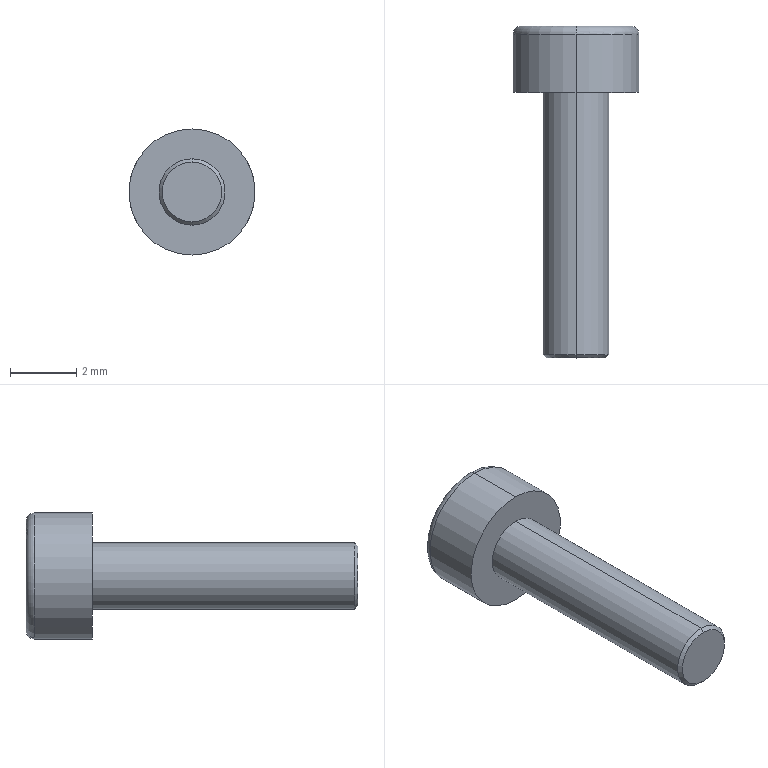Component | SolidWorks | hexagon socket head cap screws gb-4 | 1 solid | 25 faces | box 3.8 x 10 x 3.8 mm | volume 45 mm3 | plane 15 | cone 4 | cylinder 4 | torus 2 | commonest cylinder face diameters 2 x2 3.8 x2
STEP:
#1=COLOUR_RGB('',0.7922,0.8196,0.9333);
#2=FILL_AREA_STYLE_COLOUR('',#1);
#3=FILL_AREA_STYLE('',(#2));
#4=SURFACE_STYLE_FILL_AREA(#3);
#5=SURFACE_SIDE_STYLE('',(#4));
#6=SURFACE_STYLE_USAGE(.BOTH.,#5);
#7=PRESENTATION_STYLE_ASSIGNMENT((#6));
#8=CARTESIAN_POINT('',(1.349,0.4924,7.451));
#9=VERTEX_POINT('',#8);
#10=CARTESIAN_POINT('',(1.349,0.4924,7.522));
#11=VERTEX_POINT('',#10);
#12=CARTESIAN_POINT('',(1.349,0.4924,7.487));
#13=DIRECTION('',(0.,-1.,0.));
#14=DIRECTION('',(0.,0.,-1.));
#15=AXIS2_PLACEMENT_3D('',#12,#13,#14);
#16=CIRCLE('',#15,0.03543);
#17=EDGE_CURVE('',#9,#11,#16,.T.);
#18=ORIENTED_EDGE('',*,*,#17,.F.);
#19=CARTESIAN_POINT('',(1.349,0.4963,7.448));
#20=VERTEX_POINT('',#19);
#21=CARTESIAN_POINT('',(1.349,0.4924,7.451));
#22=DIRECTION('',(0.,0.7071,-0.7071));
#23=VECTOR('',#22,39.37);
#24=LINE('',#21,#23);
#25=EDGE_CURVE('',#9,#20,#24,.T.);
#26=ORIENTED_EDGE('',*,*,#25,.T.);
#27=CARTESIAN_POINT('',(1.349,0.4963,7.526));
#28=VERTEX_POINT('',#27);
#29=CARTESIAN_POINT('',(1.349,0.4963,7.487));
#30=DIRECTION('',(0.,1.,0.));
#31=DIRECTION('',(0.,0.,-1.));
#32=AXIS2_PLACEMENT_3D('',#29,#30,#31);
#33=CIRCLE('',#32,0.03937);
#34=EDGE_CURVE('',#28,#20,#33,.T.);
#35=ORIENTED_EDGE('',*,*,#34,.F.);
#36=CARTESIAN_POINT('',(1.349,0.4924,7.522));
#37=DIRECTION('',(0.,0.7071,0.7071));
#38=VECTOR('',#37,39.37);
#39=LINE('',#36,#38);
#40=EDGE_CURVE('',#11,#28,#39,.T.);
#41=ORIENTED_EDGE('',*,*,#40,.F.);
#42=EDGE_LOOP('',(#18,#26,#35,#41));
#43=FACE_OUTER_BOUND('',#42,.T.);
#44=CARTESIAN_POINT('',(1.349,0.4924,7.487));
#45=DIRECTION('',(0.,1.,0.));
#46=DIRECTION('',(0.,0.,1.));
#47=AXIS2_PLACEMENT_3D('',#44,#45,#46);
#48=CONICAL_SURFACE('',#47,0.03543,0.7854);
#49=ADVANCED_FACE('',(#43),#48,.T.);
#50=CARTESIAN_POINT('',(1.349,0.8861,7.552));
#51=VERTEX_POINT('',#50);
#52=CARTESIAN_POINT('',(1.349,0.8861,7.422));
#53=VERTEX_POINT('',#52);
#54=CARTESIAN_POINT('',(1.349,0.8861,7.487));
#55=DIRECTION('',(0.,1.,0.));
#56=DIRECTION('',(0.,0.,-1.));
#57=AXIS2_PLACEMENT_3D('',#54,#55,#56);
#58=CIRCLE('',#57,0.06496);
#59=EDGE_CURVE('',#51,#53,#58,.T.);
#60=ORIENTED_EDGE('',*,*,#59,.F.);
#61=CARTESIAN_POINT('',(1.349,0.8762,7.562));
#62=VERTEX_POINT('',#61);
#63=CARTESIAN_POINT('',(1.349,0.8762,7.552));
#64=DIRECTION('',(1.,0.,-0.));
#65=DIRECTION('',(0.,0.,-1.));
#66=AXIS2_PLACEMENT_3D('',#63,#64,#65);
#67=CIRCLE('',#66,0.009843);
#68=EDGE_CURVE('',#51,#62,#67,.T.);
#69=ORIENTED_EDGE('',*,*,#68,.T.);
#70=CARTESIAN_POINT('',(1.349,0.8762,7.412));
#71=VERTEX_POINT('',#70);
#72=CARTESIAN_POINT('',(1.349,0.8762,7.487));
#73=DIRECTION('',(0.,-1.,0.));
#74=DIRECTION('',(0.,0.,-1.));
#75=AXIS2_PLACEMENT_3D('',#72,#73,#74);
#76=CIRCLE('',#75,0.0748);
#77=EDGE_CURVE('',#71,#62,#76,.T.);
#78=ORIENTED_EDGE('',*,*,#77,.F.);
#79=CARTESIAN_POINT('',(1.349,0.8762,7.422));
#80=DIRECTION('',(-1.,0.,0.));
#81=DIRECTION('',(0.,0.,1.));
#82=AXIS2_PLACEMENT_3D('',#79,#80,#81);
#83=CIRCLE('',#82,0.009843);
#84=EDGE_CURVE('',#53,#71,#83,.T.);
#85=ORIENTED_EDGE('',*,*,#84,.F.);
#86=EDGE_LOOP('',(#60,#69,#78,#85));
#87=FACE_OUTER_BOUND('',#86,.T.);
#88=CARTESIAN_POINT('',(1.349,0.8762,7.487));
#89=DIRECTION('',(0.,-1.,0.));
#90=DIRECTION('',(0.,0.,-1.));
#91=AXIS2_PLACEMENT_3D('',#88,#89,#90);
#92=TOROIDAL_SURFACE('',#91,0.06496,0.009843);
#93=ADVANCED_FACE('',(#87),#92,.T.);
#94=CARTESIAN_POINT('',(1.349,0.8297,7.487));
#95=VERTEX_POINT('',#94);
#96=CARTESIAN_POINT('',(1.349,0.8467,7.516));
#97=VERTEX_POINT('',#96);
#98=CARTESIAN_POINT('',(1.349,0.8467,7.516));
#99=DIRECTION('',(0.,0.5,0.866));
#100=VECTOR('',#99,39.37);
#101=LINE('',#98,#100);
#102=EDGE_CURVE('',#95,#97,#101,.T.);
#103=ORIENTED_EDGE('',*,*,#102,.F.);
#104=CARTESIAN_POINT('',(1.349,0.8467,7.457));
#105=VERTEX_POINT('',#104);
#106=CARTESIAN_POINT('',(1.349,0.8467,7.457));
#107=DIRECTION('',(0.,0.5,-0.866));
#108=VECTOR('',#107,39.37);
#109=LINE('',#106,#108);
#110=EDGE_CURVE('',#95,#105,#109,.T.);
#111=ORIENTED_EDGE('',*,*,#110,.T.);
#112=CARTESIAN_POINT('',(1.334,0.8467,7.461));
#113=VERTEX_POINT('',#112);
#114=CARTESIAN_POINT('',(1.349,0.8467,7.487));
#115=DIRECTION('',(0.,1.,0.));
#116=DIRECTION('',(0.,0.,-1.));
#117=AXIS2_PLACEMENT_3D('',#114,#115,#116);
#118=CIRCLE('',#117,0.02953);
#119=EDGE_CURVE('',#105,#113,#118,.T.);
#120=ORIENTED_EDGE('',*,*,#119,.T.);
#121=CARTESIAN_POINT('',(1.32,0.8467,7.487));
#122=VERTEX_POINT('',#121);
#123=CARTESIAN_POINT('',(1.349,0.8467,7.487));
#124=DIRECTION('',(0.,1.,0.));
#125=DIRECTION('',(0.,0.,-1.));
#126=AXIS2_PLACEMENT_3D('',#123,#124,#125);
#127=CIRCLE('',#126,0.02953);
#128=EDGE_CURVE('',#113,#122,#127,.T.);
#129=ORIENTED_EDGE('',*,*,#128,.T.);
#130=CARTESIAN_POINT('',(1.334,0.8467,7.512));
#131=VERTEX_POINT('',#130);
#132=CARTESIAN_POINT('',(1.349,0.8467,7.487));
#133=DIRECTION('',(0.,1.,0.));
#134=DIRECTION('',(0.,0.,-1.));
#135=AXIS2_PLACEMENT_3D('',#132,#133,#134);
#136=CIRCLE('',#135,0.02953);
#137=EDGE_CURVE('',#122,#131,#136,.T.);
#138=ORIENTED_EDGE('',*,*,#137,.T.);
#139=CARTESIAN_POINT('',(1.349,0.8467,7.487));
#140=DIRECTION('',(0.,1.,0.));
#141=DIRECTION('',(0.,0.,-1.));
#142=AXIS2_PLACEMENT_3D('',#139,#140,#141);
#143=CIRCLE('',#142,0.02953);
#144=EDGE_CURVE('',#131,#97,#143,.T.);
#145=ORIENTED_EDGE('',*,*,#144,.T.);
#146=EDGE_LOOP('',(#103,#111,#120,#129,#138,#145));
#147=FACE_OUTER_BOUND('',#146,.T.);
#148=CARTESIAN_POINT('',(1.349,0.8467,7.487));
#149=DIRECTION('',(0.,1.,0.));
#150=DIRECTION('',(0.,0.,1.));
#151=AXIS2_PLACEMENT_3D('',#148,#149,#150);
#152=CONICAL_SURFACE('',#151,0.02953,1.047);
#153=ADVANCED_FACE('',(#147),#152,.F.);
#154=ORIENTED_EDGE('',*,*,#34,.T.);
#155=CARTESIAN_POINT('',(1.349,0.8073,7.448));
#156=VERTEX_POINT('',#155);
#157=CARTESIAN_POINT('',(1.349,0.4924,7.448));
#158=DIRECTION('',(0.,1.,0.));
#159=VECTOR('',#158,39.37);
#160=LINE('',#157,#159);
#161=EDGE_CURVE('',#20,#156,#160,.T.);
#162=ORIENTED_EDGE('',*,*,#161,.T.);
#163=CARTESIAN_POINT('',(1.349,0.8073,7.526));
#164=VERTEX_POINT('',#163);
#165=CARTESIAN_POINT('',(1.349,0.8073,7.487));
#166=DIRECTION('',(0.,-1.,0.));
#167=DIRECTION('',(0.,0.,-1.));
#168=AXIS2_PLACEMENT_3D('',#165,#166,#167);
#169=CIRCLE('',#168,0.03937);
#170=EDGE_CURVE('',#156,#164,#169,.T.);
#171=ORIENTED_EDGE('',*,*,#170,.T.);
#172=CARTESIAN_POINT('',(1.349,0.4924,7.526));
#173=DIRECTION('',(0.,1.,0.));
#174=VECTOR('',#173,39.37);
#175=LINE('',#172,#174);
#176=EDGE_CURVE('',#28,#164,#175,.T.);
#177=ORIENTED_EDGE('',*,*,#176,.F.);
#178=EDGE_LOOP('',(#154,#162,#171,#177));
#179=FACE_OUTER_BOUND('',#178,.T.);
#180=CARTESIAN_POINT('',(1.349,0.4924,7.487));
#181=DIRECTION('',(0.,1.,0.));
#182=DIRECTION('',(0.,0.,1.));
#183=AXIS2_PLACEMENT_3D('',#180,#181,#182);
#184=CYLINDRICAL_SURFACE('',#183,0.03937);
#185=ADVANCED_FACE('',(#179),#184,.T.);
#186=CARTESIAN_POINT('',(1.349,0.8073,7.412));
#187=VERTEX_POINT('',#186);
#188=CARTESIAN_POINT('',(1.349,0.8073,7.562));
#189=VERTEX_POINT('',#188);
#190=CARTESIAN_POINT('',(1.349,0.8073,7.487));
#191=DIRECTION('',(0.,-1.,0.));
#192=DIRECTION('',(0.,0.,-1.));
#193=AXIS2_PLACEMENT_3D('',#190,#191,#192);
#194=CIRCLE('',#193,0.0748);
#195=EDGE_CURVE('',#187,#189,#194,.T.);
#196=ORIENTED_EDGE('',*,*,#195,.F.);
#197=CARTESIAN_POINT('',(1.349,0.8073,7.412));
#198=DIRECTION('',(0.,1.,0.));
#199=VECTOR('',#198,39.37);
#200=LINE('',#197,#199);
#201=EDGE_CURVE('',#187,#71,#200,.T.);
#202=ORIENTED_EDGE('',*,*,#201,.T.);
#203=ORIENTED_EDGE('',*,*,#77,.T.);
#204=CARTESIAN_POINT('',(1.349,0.8073,7.562));
#205=DIRECTION('',(0.,1.,0.));
#206=VECTOR('',#205,39.37);
#207=LINE('',#204,#206);
#208=EDGE_CURVE('',#189,#62,#207,.T.);
#209=ORIENTED_EDGE('',*,*,#208,.F.);
#210=EDGE_LOOP('',(#196,#202,#203,#209));
#211=FACE_OUTER_BOUND('',#210,.T.);
#212=CARTESIAN_POINT('',(1.349,0.8073,7.487));
#213=DIRECTION('',(0.,1.,0.));
#214=DIRECTION('',(0.,0.,1.));
#215=AXIS2_PLACEMENT_3D('',#212,#213,#214);
#216=CYLINDRICAL_SURFACE('',#215,0.0748);
#217=ADVANCED_FACE('',(#211),#216,.T.);
#218=ORIENTED_EDGE('',*,*,#128,.F.);
#219=CARTESIAN_POINT('',(1.32,0.8467,7.47));
#220=VERTEX_POINT('',#219);
#221=CARTESIAN_POINT('',(1.32,0.8467,7.47));
#222=DIRECTION('',(0.866,0.,-0.5));
#223=VECTOR('',#222,39.37);
#224=LINE('',#221,#223);
#225=EDGE_CURVE('',#220,#113,#224,.T.);
#226=ORIENTED_EDGE('',*,*,#225,.F.);
#227=CARTESIAN_POINT('',(1.32,0.8467,7.504));
#228=DIRECTION('',(-0.,0.,-1.));
#229=VECTOR('',#228,39.37);
#230=LINE('',#227,#229);
#231=EDGE_CURVE('',#122,#220,#230,.T.);
#232=ORIENTED_EDGE('',*,*,#231,.F.);
#233=EDGE_LOOP('',(#218,#226,#232));
#234=FACE_OUTER_BOUND('',#233,.T.);
#235=CARTESIAN_POINT('',(1.349,0.8467,7.453));
#236=DIRECTION('',(0.,-1.,0.));
#237=DIRECTION('',(0.,0.,-1.));
#238=AXIS2_PLACEMENT_3D('',#235,#236,#237);
#239=PLANE('',#238);
#240=ADVANCED_FACE('',(#234),#239,.F.);
#241=ORIENTED_EDGE('',*,*,#137,.F.);
#242=CARTESIAN_POINT('',(1.32,0.8467,7.504));
#243=VERTEX_POINT('',#242);
#244=CARTESIAN_POINT('',(1.32,0.8467,7.504));
#245=DIRECTION('',(-0.,0.,-1.));
#246=VECTOR('',#245,39.37);
#247=LINE('',#244,#246);
#248=EDGE_CURVE('',#243,#122,#247,.T.);
#249=ORIENTED_EDGE('',*,*,#248,.F.);
#250=CARTESIAN_POINT('',(1.349,0.8467,7.521));
#251=DIRECTION('',(-0.866,0.,-0.5));
#252=VECTOR('',#251,39.37);
#253=LINE('',#250,#252);
#254=EDGE_CURVE('',#131,#243,#253,.T.);
#255=ORIENTED_EDGE('',*,*,#254,.F.);
#256=EDGE_LOOP('',(#241,#249,#255));
#257=FACE_OUTER_BOUND('',#256,.T.);
#258=CARTESIAN_POINT('',(1.349,0.8467,7.453));
#259=DIRECTION('',(0.,-1.,0.));
#260=DIRECTION('',(0.,0.,-1.));
#261=AXIS2_PLACEMENT_3D('',#258,#259,#260);
#262=PLANE('',#261);
#263=ADVANCED_FACE('',(#257),#262,.F.);
#264=ORIENTED_EDGE('',*,*,#144,.F.);
#265=CARTESIAN_POINT('',(1.349,0.8467,7.521));
#266=VERTEX_POINT('',#265);
#267=CARTESIAN_POINT('',(1.349,0.8467,7.521));
#268=DIRECTION('',(-0.866,0.,-0.5));
#269=VECTOR('',#268,39.37);
#270=LINE('',#267,#269);
#271=EDGE_CURVE('',#266,#131,#270,.T.);
#272=ORIENTED_EDGE('',*,*,#271,.F.);
#273=CARTESIAN_POINT('',(1.364,0.8467,7.512));
#274=VERTEX_POINT('',#273);
#275=CARTESIAN_POINT('',(1.379,0.8467,7.504));
#276=DIRECTION('',(-0.866,0.,0.5));
#277=VECTOR('',#276,39.37);
#278=LINE('',#275,#277);
#279=EDGE_CURVE('',#274,#266,#278,.T.);
#280=ORIENTED_EDGE('',*,*,#279,.F.);
#281=CARTESIAN_POINT('',(1.349,0.8467,7.487));
#282=DIRECTION('',(0.,1.,0.));
#283=DIRECTION('',(0.,0.,-1.));
#284=AXIS2_PLACEMENT_3D('',#281,#282,#283);
#285=CIRCLE('',#284,0.02953);
#286=EDGE_CURVE('',#97,#274,#285,.T.);
#287=ORIENTED_EDGE('',*,*,#286,.F.);
#288=EDGE_LOOP('',(#264,#272,#280,#287));
#289=FACE_OUTER_BOUND('',#288,.T.);
#290=CARTESIAN_POINT('',(1.349,0.8467,7.453));
#291=DIRECTION('',(0.,-1.,0.));
#292=DIRECTION('',(0.,0.,-1.));
#293=AXIS2_PLACEMENT_3D('',#290,#291,#292);
#294=PLANE('',#293);
#295=ADVANCED_FACE('',(#289),#294,.F.);
#296=CARTESIAN_POINT('',(1.379,0.8467,7.487));
#297=VERTEX_POINT('',#296);
#298=CARTESIAN_POINT('',(1.349,0.8467,7.487));
#299=DIRECTION('',(0.,1.,0.));
#300=DIRECTION('',(0.,0.,-1.));
#301=AXIS2_PLACEMENT_3D('',#298,#299,#300);
#302=CIRCLE('',#301,0.02953);
#303=EDGE_CURVE('',#274,#297,#302,.T.);
#304=ORIENTED_EDGE('',*,*,#303,.F.);
#305=CARTESIAN_POINT('',(1.379,0.8467,7.504));
#306=VERTEX_POINT('',#305);
#307=CARTESIAN_POINT('',(1.379,0.8467,7.504));
#308=DIRECTION('',(-0.866,0.,0.5));
#309=VECTOR('',#308,39.37);
#310=LINE('',#307,#309);
#311=EDGE_CURVE('',#306,#274,#310,.T.);
#312=ORIENTED_EDGE('',*,*,#311,.F.);
#313=CARTESIAN_POINT('',(1.379,0.8467,7.47));
#314=DIRECTION('',(0.,0.,1.));
#315=VECTOR('',#314,39.37);
#316=LINE('',#313,#315);
#317=EDGE_CURVE('',#297,#306,#316,.T.);
#318=ORIENTED_EDGE('',*,*,#317,.F.);
#319=EDGE_LOOP('',(#304,#312,#318));
#320=FACE_OUTER_BOUND('',#319,.T.);
#321=CARTESIAN_POINT('',(1.349,0.8467,7.453));
#322=DIRECTION('',(0.,-1.,0.));
#323=DIRECTION('',(0.,0.,-1.));
#324=AXIS2_PLACEMENT_3D('',#321,#322,#323);
#325=PLANE('',#324);
#326=ADVANCED_FACE('',(#320),#325,.F.);
#327=CARTESIAN_POINT('',(1.364,0.8467,7.461));
#328=VERTEX_POINT('',#327);
#329=CARTESIAN_POINT('',(1.349,0.8467,7.487));
#330=DIRECTION('',(0.,-1.,0.));
#331=DIRECTION('',(0.,0.,-1.));
#332=AXIS2_PLACEMENT_3D('',#329,#330,#331);
#333=CIRCLE('',#332,0.02953);
#334=EDGE_CURVE('',#328,#297,#333,.T.);
#335=ORIENTED_EDGE('',*,*,#334,.T.);
#336=CARTESIAN_POINT('',(1.379,0.8467,7.47));
#337=VERTEX_POINT('',#336);
#338=CARTESIAN_POINT('',(1.379,0.8467,7.47));
#339=DIRECTION('',(0.,0.,1.));
#340=VECTOR('',#339,39.37);
#341=LINE('',#338,#340);
#342=EDGE_CURVE('',#337,#297,#341,.T.);
#343=ORIENTED_EDGE('',*,*,#342,.F.);
#344=CARTESIAN_POINT('',(1.349,0.8467,7.453));
#345=DIRECTION('',(0.866,0.,0.5));
#346=VECTOR('',#345,39.37);
#347=LINE('',#344,#346);
#348=EDGE_CURVE('',#328,#337,#347,.T.);
#349=ORIENTED_EDGE('',*,*,#348,.F.);
#350=EDGE_LOOP('',(#335,#343,#349));
#351=FACE_OUTER_BOUND('',#350,.T.);
#352=CARTESIAN_POINT('',(1.349,0.8467,7.453));
#353=DIRECTION('',(0.,-1.,0.));
#354=DIRECTION('',(0.,0.,-1.));
#355=AXIS2_PLACEMENT_3D('',#352,#353,#354);
#356=PLANE('',#355);
#357=ADVANCED_FACE('',(#351),#356,.F.);
#358=CARTESIAN_POINT('',(1.349,0.8467,7.487));
#359=DIRECTION('',(0.,1.,0.));
#360=DIRECTION('',(0.,0.,-1.));
#361=AXIS2_PLACEMENT_3D('',#358,#359,#360);
#362=CIRCLE('',#361,0.02953);
#363=EDGE_CURVE('',#328,#105,#362,.T.);
#364=ORIENTED_EDGE('',*,*,#363,.F.);
#365=CARTESIAN_POINT('',(1.349,0.8467,7.453));
#366=VERTEX_POINT('',#365);
#367=CARTESIAN_POINT('',(1.349,0.8467,7.453));
#368=DIRECTION('',(0.866,0.,0.5));
#369=VECTOR('',#368,39.37);
#370=LINE('',#367,#369);
#371=EDGE_CURVE('',#366,#328,#370,.T.);
#372=ORIENTED_EDGE('',*,*,#371,.F.);
#373=CARTESIAN_POINT('',(1.32,0.8467,7.47));
#374=DIRECTION('',(0.866,0.,-0.5));
#375=VECTOR('',#374,39.37);
#376=LINE('',#373,#375);
#377=EDGE_CURVE('',#113,#366,#376,.T.);
#378=ORIENTED_EDGE('',*,*,#377,.F.);
#379=ORIENTED_EDGE('',*,*,#119,.F.);
#380=EDGE_LOOP('',(#364,#372,#378,#379));
#381=FACE_OUTER_BOUND('',#380,.T.);
#382=CARTESIAN_POINT('',(1.349,0.8467,7.453));
#383=DIRECTION('',(0.,-1.,0.));
#384=DIRECTION('',(0.,0.,-1.));
#385=AXIS2_PLACEMENT_3D('',#382,#383,#384);
#386=PLANE('',#385);
#387=ADVANCED_FACE('',(#381),#386,.F.);
#388=CARTESIAN_POINT('',(1.349,0.8861,7.487));
#389=DIRECTION('',(0.,1.,0.));
#390=DIRECTION('',(0.,0.,-1.));
#391=AXIS2_PLACEMENT_3D('',#388,#389,#390);
#392=CIRCLE('',#391,0.06496);
#393=EDGE_CURVE('',#53,#51,#392,.T.);
#394=ORIENTED_EDGE('',*,*,#393,.T.);
#395=ORIENTED_EDGE('',*,*,#59,.T.);
#396=EDGE_LOOP('',(#394,#395));
#397=FACE_OUTER_BOUND('',#396,.T.);
#398=CARTESIAN_POINT('',(1.32,0.8861,7.47));
#399=VERTEX_POINT('',#398);
#400=CARTESIAN_POINT('',(1.349,0.8861,7.453));
#401=VERTEX_POINT('',#400);
#402=CARTESIAN_POINT('',(1.32,0.8861,7.47));
#403=DIRECTION('',(0.866,0.,-0.5));
#404=VECTOR('',#403,39.37);
#405=LINE('',#402,#404);
#406=EDGE_CURVE('',#399,#401,#405,.T.);
#407=ORIENTED_EDGE('',*,*,#406,.T.);
#408=CARTESIAN_POINT('',(1.379,0.8861,7.47));
#409=VERTEX_POINT('',#408);
#410=CARTESIAN_POINT('',(1.349,0.8861,7.453));
#411=DIRECTION('',(0.866,0.,0.5));
#412=VECTOR('',#411,39.37);
#413=LINE('',#410,#412);
#414=EDGE_CURVE('',#401,#409,#413,.T.);
#415=ORIENTED_EDGE('',*,*,#414,.T.);
#416=CARTESIAN_POINT('',(1.379,0.8861,7.504));
#417=VERTEX_POINT('',#416);
#418=CARTESIAN_POINT('',(1.379,0.8861,7.47));
#419=DIRECTION('',(0.,0.,1.));
#420=VECTOR('',#419,39.37);
#421=LINE('',#418,#420);
#422=EDGE_CURVE('',#409,#417,#421,.T.);
#423=ORIENTED_EDGE('',*,*,#422,.T.);
#424=CARTESIAN_POINT('',(1.349,0.8861,7.521));
#425=VERTEX_POINT('',#424);
#426=CARTESIAN_POINT('',(1.379,0.8861,7.504));
#427=DIRECTION('',(-0.866,0.,0.5));
#428=VECTOR('',#427,39.37);
#429=LINE('',#426,#428);
#430=EDGE_CURVE('',#417,#425,#429,.T.);
#431=ORIENTED_EDGE('',*,*,#430,.T.);
#432=CARTESIAN_POINT('',(1.32,0.8861,7.504));
#433=VERTEX_POINT('',#432);
#434=CARTESIAN_POINT('',(1.349,0.8861,7.521));
#435=DIRECTION('',(-0.866,0.,-0.5));
#436=VECTOR('',#435,39.37);
#437=LINE('',#434,#436);
#438=EDGE_CURVE('',#425,#433,#437,.T.);
#439=ORIENTED_EDGE('',*,*,#438,.T.);
#440=CARTESIAN_POINT('',(1.32,0.8861,7.504));
#441=DIRECTION('',(-0.,0.,-1.));
#442=VECTOR('',#441,39.37);
#443=LINE('',#440,#442);
#444=EDGE_CURVE('',#433,#399,#443,.T.);
#445=ORIENTED_EDGE('',*,*,#444,.T.);
#446=EDGE_LOOP('',(#407,#415,#423,#431,#439,#445));
#447=FACE_BOUND('',#446,.T.);
#448=CARTESIAN_POINT('',(1.349,0.8861,7.487));
#449=DIRECTION('',(0.,-1.,0.));
#450=DIRECTION('',(0.,0.,-1.));
#451=AXIS2_PLACEMENT_3D('',#448,#449,#450);
#452=PLANE('',#451);
#453=ADVANCED_FACE('',(#397,#447),#452,.F.);
#454=CARTESIAN_POINT('',(1.349,0.8073,7.487));
#455=DIRECTION('',(0.,-1.,0.));
#456=DIRECTION('',(0.,0.,-1.));
#457=AXIS2_PLACEMENT_3D('',#454,#455,#456);
#458=CIRCLE('',#457,0.0748);
#459=EDGE_CURVE('',#189,#187,#458,.T.);
#460=ORIENTED_EDGE('',*,*,#459,.T.);
#461=ORIENTED_EDGE('',*,*,#195,.T.);
#462=EDGE_LOOP('',(#460,#461));
#463=FACE_OUTER_BOUND('',#462,.T.);
#464=CARTESIAN_POINT('',(1.349,0.8073,7.487));
#465=DIRECTION('',(0.,-1.,0.));
#466=DIRECTION('',(0.,0.,-1.));
#467=AXIS2_PLACEMENT_3D('',#464,#465,#466);
#468=CIRCLE('',#467,0.03937);
#469=EDGE_CURVE('',#164,#156,#468,.T.);
#470=ORIENTED_EDGE('',*,*,#469,.F.);
#471=ORIENTED_EDGE('',*,*,#170,.F.);
#472=EDGE_LOOP('',(#470,#471));
#473=FACE_BOUND('',#472,.T.);
#474=CARTESIAN_POINT('',(1.349,0.8073,7.487));
#475=DIRECTION('',(0.,-1.,0.));
#476=DIRECTION('',(0.,0.,-1.));
#477=AXIS2_PLACEMENT_3D('',#474,#475,#476);
#478=PLANE('',#477);
#479=ADVANCED_FACE('',(#463,#473),#478,.T.);
#480=ORIENTED_EDGE('',*,*,#201,.F.);
#481=ORIENTED_EDGE('',*,*,#459,.F.);
#482=ORIENTED_EDGE('',*,*,#208,.T.);
#483=CARTESIAN_POINT('',(1.349,0.8762,7.487));
#484=DIRECTION('',(0.,-1.,0.));
#485=DIRECTION('',(0.,0.,-1.));
#486=AXIS2_PLACEMENT_3D('',#483,#484,#485);
#487=CIRCLE('',#486,0.0748);
#488=EDGE_CURVE('',#62,#71,#487,.T.);
#489=ORIENTED_EDGE('',*,*,#488,.T.);
#490=EDGE_LOOP('',(#480,#481,#482,#489));
#491=FACE_OUTER_BOUND('',#490,.T.);
#492=CARTESIAN_POINT('',(1.349,0.8073,7.487));
#493=DIRECTION('',(0.,1.,0.));
#494=DIRECTION('',(0.,0.,1.));
#495=AXIS2_PLACEMENT_3D('',#492,#493,#494);
#496=CYLINDRICAL_SURFACE('',#495,0.0748);
#497=ADVANCED_FACE('',(#491),#496,.T.);
#498=ORIENTED_EDGE('',*,*,#161,.F.);
#499=CARTESIAN_POINT('',(1.349,0.4963,7.487));
#500=DIRECTION('',(0.,1.,0.));
#501=DIRECTION('',(0.,0.,-1.));
#502=AXIS2_PLACEMENT_3D('',#499,#500,#501);
#503=CIRCLE('',#502,0.03937);
#504=EDGE_CURVE('',#20,#28,#503,.T.);
#505=ORIENTED_EDGE('',*,*,#504,.T.);
#506=ORIENTED_EDGE('',*,*,#176,.T.);
#507=ORIENTED_EDGE('',*,*,#469,.T.);
#508=EDGE_LOOP('',(#498,#505,#506,#507));
#509=FACE_OUTER_BOUND('',#508,.T.);
#510=CARTESIAN_POINT('',(1.349,0.4924,7.487));
#511=DIRECTION('',(0.,1.,0.));
#512=DIRECTION('',(0.,0.,1.));
#513=AXIS2_PLACEMENT_3D('',#510,#511,#512);
#514=CYLINDRICAL_SURFACE('',#513,0.03937);
#515=ADVANCED_FACE('',(#509),#514,.T.);
#516=CARTESIAN_POINT('',(1.349,0.4924,7.487));
#517=DIRECTION('',(0.,-1.,0.));
#518=DIRECTION('',(0.,0.,-1.));
#519=AXIS2_PLACEMENT_3D('',#516,#517,#518);
#520=CIRCLE('',#519,0.03543);
#521=EDGE_CURVE('',#11,#9,#520,.T.);
#522=ORIENTED_EDGE('',*,*,#521,.T.);
#523=ORIENTED_EDGE('',*,*,#17,.T.);
#524=EDGE_LOOP('',(#522,#523));
#525=FACE_OUTER_BOUND('',#524,.T.);
#526=CARTESIAN_POINT('',(1.349,0.4924,7.487));
#527=DIRECTION('',(0.,-1.,0.));
#528=DIRECTION('',(0.,0.,-1.));
#529=AXIS2_PLACEMENT_3D('',#526,#527,#528);
#530=PLANE('',#529);
#531=ADVANCED_FACE('',(#525),#530,.T.);
#532=ORIENTED_EDGE('',*,*,#406,.F.);
#533=CARTESIAN_POINT('',(1.32,0.8467,7.47));
#534=DIRECTION('',(0.,1.,0.));
#535=VECTOR('',#534,39.37);
#536=LINE('',#533,#535);
#537=EDGE_CURVE('',#220,#399,#536,.T.);
#538=ORIENTED_EDGE('',*,*,#537,.F.);
#539=ORIENTED_EDGE('',*,*,#225,.T.);
#540=ORIENTED_EDGE('',*,*,#377,.T.);
#541=CARTESIAN_POINT('',(1.349,0.8467,7.453));
#542=DIRECTION('',(0.,1.,0.));
#543=VECTOR('',#542,39.37);
#544=LINE('',#541,#543);
#545=EDGE_CURVE('',#366,#401,#544,.T.);
#546=ORIENTED_EDGE('',*,*,#545,.T.);
#547=EDGE_LOOP('',(#532,#538,#539,#540,#546));
#548=FACE_OUTER_BOUND('',#547,.T.);
#549=CARTESIAN_POINT('',(1.32,0.8467,7.47));
#550=DIRECTION('',(0.5,0.,0.866));
#551=DIRECTION('',(-0.866,0.,0.5));
#552=AXIS2_PLACEMENT_3D('',#549,#550,#551);
#553=PLANE('',#552);
#554=ADVANCED_FACE('',(#548),#553,.T.);
#555=ORIENTED_EDGE('',*,*,#414,.F.);
#556=ORIENTED_EDGE('',*,*,#545,.F.);
#557=ORIENTED_EDGE('',*,*,#371,.T.);
#558=ORIENTED_EDGE('',*,*,#348,.T.);
#559=CARTESIAN_POINT('',(1.379,0.8467,7.47));
#560=DIRECTION('',(0.,1.,0.));
#561=VECTOR('',#560,39.37);
#562=LINE('',#559,#561);
#563=EDGE_CURVE('',#337,#409,#562,.T.);
#564=ORIENTED_EDGE('',*,*,#563,.T.);
#565=EDGE_LOOP('',(#555,#556,#557,#558,#564));
#566=FACE_OUTER_BOUND('',#565,.T.);
#567=CARTESIAN_POINT('',(1.349,0.8467,7.453));
#568=DIRECTION('',(-0.5,0.,0.866));
#569=DIRECTION('',(-0.866,0.,-0.5));
#570=AXIS2_PLACEMENT_3D('',#567,#568,#569);
#571=PLANE('',#570);
#572=ADVANCED_FACE('',(#566),#571,.T.);
#573=ORIENTED_EDGE('',*,*,#422,.F.);
#574=ORIENTED_EDGE('',*,*,#563,.F.);
#575=ORIENTED_EDGE('',*,*,#342,.T.);
#576=ORIENTED_EDGE('',*,*,#317,.T.);
#577=CARTESIAN_POINT('',(1.379,0.8467,7.504));
#578=DIRECTION('',(0.,1.,0.));
#579=VECTOR('',#578,39.37);
#580=LINE('',#577,#579);
#581=EDGE_CURVE('',#306,#417,#580,.T.);
#582=ORIENTED_EDGE('',*,*,#581,.T.);
#583=EDGE_LOOP('',(#573,#574,#575,#576,#582));
#584=FACE_OUTER_BOUND('',#583,.T.);
#585=CARTESIAN_POINT('',(1.379,0.8467,7.47));
#586=DIRECTION('',(-1.,0.,0.));
#587=DIRECTION('',(0.,0.,-1.));
#588=AXIS2_PLACEMENT_3D('',#585,#586,#587);
#589=PLANE('',#588);
#590=ADVANCED_FACE('',(#584),#589,.T.);
#591=ORIENTED_EDGE('',*,*,#430,.F.);
#592=ORIENTED_EDGE('',*,*,#581,.F.);
#593=ORIENTED_EDGE('',*,*,#311,.T.);
#594=ORIENTED_EDGE('',*,*,#279,.T.);
#595=CARTESIAN_POINT('',(1.349,0.8467,7.521));
#596=DIRECTION('',(0.,1.,0.));
#597=VECTOR('',#596,39.37);
#598=LINE('',#595,#597);
#599=EDGE_CURVE('',#266,#425,#598,.T.);
#600=ORIENTED_EDGE('',*,*,#599,.T.);
#601=EDGE_LOOP('',(#591,#592,#593,#594,#600));
#602=FACE_OUTER_BOUND('',#601,.T.);
#603=CARTESIAN_POINT('',(1.379,0.8467,7.504));
#604=DIRECTION('',(-0.5,0.,-0.866));
#605=DIRECTION('',(0.866,0.,-0.5));
#606=AXIS2_PLACEMENT_3D('',#603,#604,#605);
#607=PLANE('',#606);
#608=ADVANCED_FACE('',(#602),#607,.T.);
#609=ORIENTED_EDGE('',*,*,#438,.F.);
#610=ORIENTED_EDGE('',*,*,#599,.F.);
#611=ORIENTED_EDGE('',*,*,#271,.T.);
#612=ORIENTED_EDGE('',*,*,#254,.T.);
#613=CARTESIAN_POINT('',(1.32,0.8467,7.504));
#614=DIRECTION('',(0.,1.,0.));
#615=VECTOR('',#614,39.37);
#616=LINE('',#613,#615);
#617=EDGE_CURVE('',#243,#433,#616,.T.);
#618=ORIENTED_EDGE('',*,*,#617,.T.);
#619=EDGE_LOOP('',(#609,#610,#611,#612,#618));
#620=FACE_OUTER_BOUND('',#619,.T.);
#621=CARTESIAN_POINT('',(1.349,0.8467,7.521));
#622=DIRECTION('',(0.5,0.,-0.866));
#623=DIRECTION('',(0.866,0.,0.5));
#624=AXIS2_PLACEMENT_3D('',#621,#622,#623);
#625=PLANE('',#624);
#626=ADVANCED_FACE('',(#620),#625,.T.);
#627=ORIENTED_EDGE('',*,*,#444,.F.);
#628=ORIENTED_EDGE('',*,*,#617,.F.);
#629=ORIENTED_EDGE('',*,*,#248,.T.);
#630=ORIENTED_EDGE('',*,*,#231,.T.);
#631=ORIENTED_EDGE('',*,*,#537,.T.);
#632=EDGE_LOOP('',(#627,#628,#629,#630,#631));
#633=FACE_OUTER_BOUND('',#632,.T.);
#634=CARTESIAN_POINT('',(1.32,0.8467,7.504));
#635=DIRECTION('',(1.,0.,-0.));
#636=DIRECTION('',(0.,0.,1.));
#637=AXIS2_PLACEMENT_3D('',#634,#635,#636);
#638=PLANE('',#637);
#639=ADVANCED_FACE('',(#633),#638,.T.);
#640=ORIENTED_EDGE('',*,*,#110,.F.);
#641=ORIENTED_EDGE('',*,*,#102,.T.);
#642=ORIENTED_EDGE('',*,*,#286,.T.);
#643=ORIENTED_EDGE('',*,*,#303,.T.);
#644=ORIENTED_EDGE('',*,*,#334,.F.);
#645=ORIENTED_EDGE('',*,*,#363,.T.);
#646=EDGE_LOOP('',(#640,#641,#642,#643,#644,#645));
#647=FACE_OUTER_BOUND('',#646,.T.);
#648=CARTESIAN_POINT('',(1.349,0.8467,7.487));
#649=DIRECTION('',(0.,1.,0.));
#650=DIRECTION('',(0.,0.,1.));
#651=AXIS2_PLACEMENT_3D('',#648,#649,#650);
#652=CONICAL_SURFACE('',#651,0.02953,1.047);
#653=ADVANCED_FACE('',(#647),#652,.F.);
#654=ORIENTED_EDGE('',*,*,#68,.F.);
#655=ORIENTED_EDGE('',*,*,#393,.F.);
#656=ORIENTED_EDGE('',*,*,#84,.T.);
#657=ORIENTED_EDGE('',*,*,#488,.F.);
#658=EDGE_LOOP('',(#654,#655,#656,#657));
#659=FACE_OUTER_BOUND('',#658,.T.);
#660=CARTESIAN_POINT('',(1.349,0.8762,7.487));
#661=DIRECTION('',(0.,-1.,0.));
#662=DIRECTION('',(0.,0.,-1.));
#663=AXIS2_PLACEMENT_3D('',#660,#661,#662);
#664=TOROIDAL_SURFACE('',#663,0.06496,0.009843);
#665=ADVANCED_FACE('',(#659),#664,.T.);
#666=ORIENTED_EDGE('',*,*,#25,.F.);
#667=ORIENTED_EDGE('',*,*,#521,.F.);
#668=ORIENTED_EDGE('',*,*,#40,.T.);
#669=ORIENTED_EDGE('',*,*,#504,.F.);
#670=EDGE_LOOP('',(#666,#667,#668,#669));
#671=FACE_OUTER_BOUND('',#670,.T.);
#672=CARTESIAN_POINT('',(1.349,0.4924,7.487));
#673=DIRECTION('',(0.,1.,0.));
#674=DIRECTION('',(0.,0.,1.));
#675=AXIS2_PLACEMENT_3D('',#672,#673,#674);
#676=CONICAL_SURFACE('',#675,0.03543,0.7854);
#677=ADVANCED_FACE('',(#671),#676,.T.);
#678=CLOSED_SHELL('',(#49,#93,#153,#185,#217,#240,#263,#295,#326,#357,#387,#453,#479,#497,#515,#531,#554,#572,#590,#608,#626,#639,#653,#665,#677));
#679=MANIFOLD_SOLID_BREP('',#678);
#680=STYLED_ITEM('',(#7),#679);
#681=PRESENTATION_LAYER_ASSIGNMENT('','',(#680));
#682=(LENGTH_UNIT()NAMED_UNIT(*)SI_UNIT($,.METRE.));
#683=LENGTH_MEASURE_WITH_UNIT(LENGTH_MEASURE(0.0254),#682);
#684=DIMENSIONAL_EXPONENTS(1.,0.,0.,0.,0.,0.,0.);
#685=(CONVERSION_BASED_UNIT('',#683)LENGTH_UNIT()NAMED_UNIT(#684));
#686=UNCERTAINTY_MEASURE_WITH_UNIT(LENGTH_MEASURE(0.00001),#685,'','');
#687=(NAMED_UNIT(*)PLANE_ANGLE_UNIT()SI_UNIT($,.RADIAN.));
#688=(NAMED_UNIT(*)SI_UNIT($,.STERADIAN.)SOLID_ANGLE_UNIT());
#689=(GEOMETRIC_REPRESENTATION_CONTEXT(3)GLOBAL_UNCERTAINTY_ASSIGNED_CONTEXT((#686))GLOBAL_UNIT_ASSIGNED_CONTEXT((#685,#687,#688))REPRESENTATION_CONTEXT('',''));
#690=MECHANICAL_DESIGN_GEOMETRIC_PRESENTATION_REPRESENTATION('',(#680),#689);
#691=CARTESIAN_POINT('',(0.,0.,0.));
#692=DIRECTION('',(0.,0.,1.));
#693=DIRECTION('',(1.,0.,0.));
#694=AXIS2_PLACEMENT_3D('',#691,#692,#693);
#695=(LENGTH_UNIT()NAMED_UNIT(*)SI_UNIT($,.METRE.));
#696=LENGTH_MEASURE_WITH_UNIT(LENGTH_MEASURE(0.0254),#695);
#697=DIMENSIONAL_EXPONENTS(1.,0.,0.,0.,0.,0.,0.);
#698=(CONVERSION_BASED_UNIT('',#696)LENGTH_UNIT()NAMED_UNIT(#697));
#699=UNCERTAINTY_MEASURE_WITH_UNIT(LENGTH_MEASURE(0.00001),#698,'','');
#700=(NAMED_UNIT(*)PLANE_ANGLE_UNIT()SI_UNIT($,.RADIAN.));
#701=(NAMED_UNIT(*)SI_UNIT($,.STERADIAN.)SOLID_ANGLE_UNIT());
#702=(GEOMETRIC_REPRESENTATION_CONTEXT(3)GLOBAL_UNCERTAINTY_ASSIGNED_CONTEXT((#699))GLOBAL_UNIT_ASSIGNED_CONTEXT((#698,#700,#701))REPRESENTATION_CONTEXT('',''));
#703=ADVANCED_BREP_SHAPE_REPRESENTATION('',(#679,#694),#702);